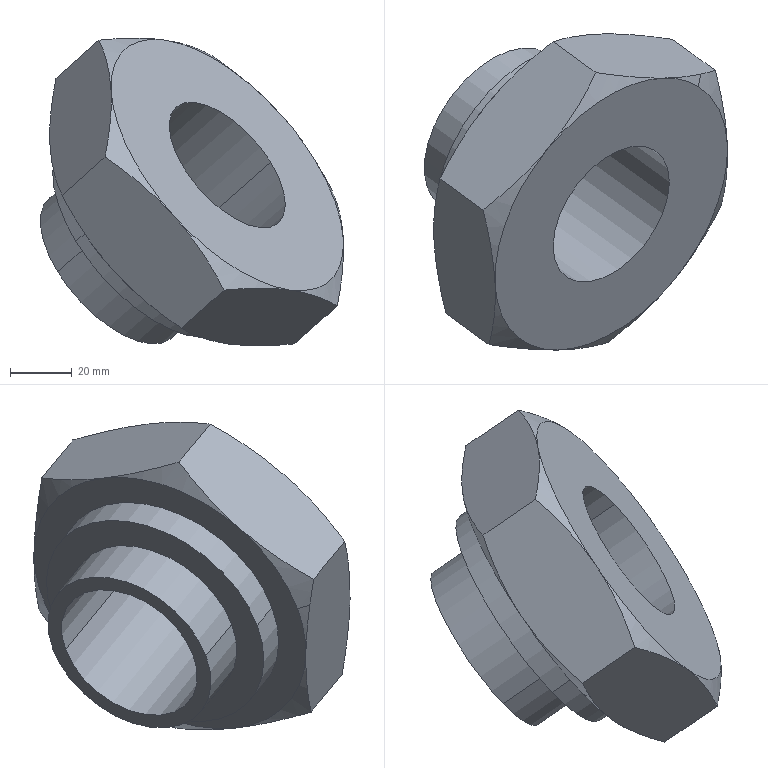Component | SolidWorks | Gasket2-1 | 1 solid | 30 faces | box 98.1 x 102.24 x 99.49 mm | volume 244481 mm3 | cone 14 | plane 10 | cylinder 6 | commonest cylinder face diameters 60 x2 50 x2 80 x2 | material Copper
STEP:
#1=COLOUR_RGB('',0.7922,0.8196,0.9333);
#2=FILL_AREA_STYLE_COLOUR('',#1);
#3=FILL_AREA_STYLE('',(#2));
#4=SURFACE_STYLE_FILL_AREA(#3);
#5=SURFACE_SIDE_STYLE('',(#4));
#6=SURFACE_STYLE_USAGE(.BOTH.,#5);
#7=PRESENTATION_STYLE_ASSIGNMENT((#6));
#8=CARTESIAN_POINT('',(6.93,-76.852,19.128));
#9=VERTEX_POINT('',#8);
#10=CARTESIAN_POINT('',(7.298,-77.585,18.111));
#11=VERTEX_POINT('',#10);
#12=CARTESIAN_POINT('',(8.409,-75.962,18.181));
#13=DIRECTION('',(0.6592,-0.4763,0.5818));
#14=DIRECTION('',(0.5643,0.8248,0.03594));
#15=AXIS2_PLACEMENT_3D('',#12,#13,#14);
#16=CIRCLE('',#15,1.969);
#17=EDGE_CURVE('',#9,#11,#16,.T.);
#18=ORIENTED_EDGE('',*,*,#17,.T.);
#19=CARTESIAN_POINT('',(7.272,-77.743,18.154));
#20=VERTEX_POINT('',#19);
#21=CARTESIAN_POINT('',(7.298,-77.585,18.111));
#22=DIRECTION('',(-0.1591,-0.9525,0.2598));
#23=VECTOR('',#22,39.37);
#24=LINE('',#21,#23);
#25=EDGE_CURVE('',#11,#20,#24,.T.);
#26=ORIENTED_EDGE('',*,*,#25,.T.);
#27=CARTESIAN_POINT('',(7.085,-77.793,18.485));
#28=VERTEX_POINT('',#27);
#29=CARTESIAN_POINT('',(7.272,-77.743,18.154));
#30=CARTESIAN_POINT('',(7.206,-77.757,18.262));
#31=CARTESIAN_POINT('',(7.144,-77.774,18.373));
#32=CARTESIAN_POINT('',(7.085,-77.793,18.485));
#33=B_SPLINE_CURVE_WITH_KNOTS('',3,(#29,#30,#31,#32),.UNSPECIFIED.,.F.,.F.,(4,4),(0.04863,0.05831),.UNSPECIFIED.);
#34=EDGE_CURVE('',#20,#28,#33,.T.);
#35=ORIENTED_EDGE('',*,*,#34,.T.);
#36=CARTESIAN_POINT('',(7.085,-77.793,18.485));
#37=CARTESIAN_POINT('',(7.043,-77.627,18.576));
#38=CARTESIAN_POINT('',(7.008,-77.464,18.673));
#39=CARTESIAN_POINT('',(6.968,-77.229,18.832));
#40=CARTESIAN_POINT('',(6.957,-77.151,18.888));
#41=CARTESIAN_POINT('',(6.94,-76.999,19.004));
#42=CARTESIAN_POINT('',(6.934,-76.925,19.065));
#43=CARTESIAN_POINT('',(6.93,-76.852,19.128));
#44=B_SPLINE_CURVE_WITH_KNOTS('',3,(#36,#37,#38,#39,#40,#41,#42,#43),.UNSPECIFIED.,.F.,.F.,(4,2,2,4),(0.00000026,0.0146,0.02191,0.02921),.UNSPECIFIED.);
#45=EDGE_CURVE('',#28,#9,#44,.T.);
#46=ORIENTED_EDGE('',*,*,#45,.T.);
#47=EDGE_LOOP('',(#18,#26,#35,#46));
#48=FACE_OUTER_BOUND('',#47,.T.);
#49=CARTESIAN_POINT('',(8.409,-75.962,18.181));
#50=DIRECTION('',(0.6592,-0.4763,0.5818));
#51=DIRECTION('',(-0.5643,-0.8248,-0.03594));
#52=AXIS2_PLACEMENT_3D('',#49,#50,#51);
#53=CONICAL_SURFACE('',#52,1.969,1.047);
#54=ADVANCED_FACE('',(#48),#53,.T.);
#55=CARTESIAN_POINT('',(10.298,-74.901,18.939));
#56=VERTEX_POINT('',#55);
#57=CARTESIAN_POINT('',(9.869,-74.794,19.513));
#58=VERTEX_POINT('',#57);
#59=CARTESIAN_POINT('',(9.188,-76.524,18.869));
#60=DIRECTION('',(0.6592,-0.4763,0.5818));
#61=DIRECTION('',(0.5643,0.8248,0.03594));
#62=AXIS2_PLACEMENT_3D('',#59,#60,#61);
#63=CIRCLE('',#62,1.969);
#64=EDGE_CURVE('',#56,#58,#63,.T.);
#65=ORIENTED_EDGE('',*,*,#64,.F.);
#66=CARTESIAN_POINT('',(10.325,-74.743,18.896));
#67=VERTEX_POINT('',#66);
#68=CARTESIAN_POINT('',(10.298,-74.901,18.939));
#69=DIRECTION('',(0.1591,0.9525,-0.2598));
#70=VECTOR('',#69,39.37);
#71=LINE('',#68,#70);
#72=EDGE_CURVE('',#56,#67,#71,.T.);
#73=ORIENTED_EDGE('',*,*,#72,.T.);
#74=CARTESIAN_POINT('',(10.325,-74.743,18.896));
#75=CARTESIAN_POINT('',(10.258,-74.758,19.005));
#76=CARTESIAN_POINT('',(10.187,-74.769,19.111));
#77=CARTESIAN_POINT('',(10.036,-74.786,19.317));
#78=CARTESIAN_POINT('',(9.955,-74.792,19.417));
#79=CARTESIAN_POINT('',(9.869,-74.794,19.513));
#80=B_SPLINE_CURVE_WITH_KNOTS('',3,(#74,#75,#76,#77,#78,#79),.UNSPECIFIED.,.F.,.F.,(4,2,4),(0.0097,0.01945,0.02921),.UNSPECIFIED.);
#81=EDGE_CURVE('',#67,#58,#80,.T.);
#82=ORIENTED_EDGE('',*,*,#81,.T.);
#83=EDGE_LOOP('',(#65,#73,#82));
#84=FACE_OUTER_BOUND('',#83,.T.);
#85=CARTESIAN_POINT('',(9.188,-76.524,18.869));
#86=DIRECTION('',(-0.6592,0.4763,-0.5818));
#87=DIRECTION('',(0.5643,0.8248,0.03594));
#88=AXIS2_PLACEMENT_3D('',#85,#86,#87);
#89=CONICAL_SURFACE('',#88,1.969,1.047);
#90=ADVANCED_FACE('',(#84),#89,.T.);
#91=CARTESIAN_POINT('',(7.029,-76.42,17.509));
#92=VERTEX_POINT('',#91);
#93=CARTESIAN_POINT('',(8.362,-74.472,17.594));
#94=VERTEX_POINT('',#93);
#95=CARTESIAN_POINT('',(7.695,-75.446,17.551));
#96=DIRECTION('',(-0.6592,0.4763,-0.5818));
#97=DIRECTION('',(-0.5643,-0.8248,-0.03594));
#98=AXIS2_PLACEMENT_3D('',#95,#96,#97);
#99=CIRCLE('',#98,1.181);
#100=EDGE_CURVE('',#92,#94,#99,.T.);
#101=ORIENTED_EDGE('',*,*,#100,.F.);
#102=CARTESIAN_POINT('',(7.483,-76.748,17.91));
#103=VERTEX_POINT('',#102);
#104=CARTESIAN_POINT('',(7.029,-76.42,17.509));
#105=DIRECTION('',(0.6592,-0.4763,0.5818));
#106=VECTOR('',#105,39.37);
#107=LINE('',#104,#106);
#108=EDGE_CURVE('',#92,#103,#107,.T.);
#109=ORIENTED_EDGE('',*,*,#108,.T.);
#110=CARTESIAN_POINT('',(8.816,-74.8,17.995));
#111=VERTEX_POINT('',#110);
#112=CARTESIAN_POINT('',(8.149,-75.774,17.952));
#113=DIRECTION('',(-0.6592,0.4763,-0.5818));
#114=DIRECTION('',(-0.5643,-0.8248,-0.03594));
#115=AXIS2_PLACEMENT_3D('',#112,#113,#114);
#116=CIRCLE('',#115,1.181);
#117=EDGE_CURVE('',#103,#111,#116,.T.);
#118=ORIENTED_EDGE('',*,*,#117,.T.);
#119=CARTESIAN_POINT('',(8.362,-74.472,17.594));
#120=DIRECTION('',(0.6592,-0.4763,0.5818));
#121=VECTOR('',#120,39.37);
#122=LINE('',#119,#121);
#123=EDGE_CURVE('',#94,#111,#122,.T.);
#124=ORIENTED_EDGE('',*,*,#123,.F.);
#125=EDGE_LOOP('',(#101,#109,#118,#124));
#126=FACE_OUTER_BOUND('',#125,.T.);
#127=CARTESIAN_POINT('',(7.695,-75.446,17.551));
#128=DIRECTION('',(0.6592,-0.4763,0.5818));
#129=DIRECTION('',(0.5643,0.8248,0.03594));
#130=AXIS2_PLACEMENT_3D('',#127,#128,#129);
#131=CYLINDRICAL_SURFACE('',#130,1.181);
#132=ADVANCED_FACE('',(#126),#131,.T.);
#133=CARTESIAN_POINT('',(8.251,-74.634,17.587));
#134=VERTEX_POINT('',#133);
#135=CARTESIAN_POINT('',(7.14,-76.258,17.516));
#136=VERTEX_POINT('',#135);
#137=CARTESIAN_POINT('',(7.695,-75.446,17.551));
#138=DIRECTION('',(-0.6592,0.4763,-0.5818));
#139=DIRECTION('',(-0.5643,-0.8248,-0.03594));
#140=AXIS2_PLACEMENT_3D('',#137,#138,#139);
#141=CIRCLE('',#140,0.9843);
#142=EDGE_CURVE('',#134,#136,#141,.T.);
#143=ORIENTED_EDGE('',*,*,#142,.T.);
#144=CARTESIAN_POINT('',(8.632,-77.336,18.833));
#145=VERTEX_POINT('',#144);
#146=CARTESIAN_POINT('',(7.14,-76.258,17.516));
#147=DIRECTION('',(0.6592,-0.4763,0.5818));
#148=VECTOR('',#147,39.37);
#149=LINE('',#146,#148);
#150=EDGE_CURVE('',#136,#145,#149,.T.);
#151=ORIENTED_EDGE('',*,*,#150,.T.);
#152=CARTESIAN_POINT('',(9.743,-75.712,18.904));
#153=VERTEX_POINT('',#152);
#154=CARTESIAN_POINT('',(9.188,-76.524,18.869));
#155=DIRECTION('',(-0.6592,0.4763,-0.5818));
#156=DIRECTION('',(-0.5643,-0.8248,-0.03594));
#157=AXIS2_PLACEMENT_3D('',#154,#155,#156);
#158=CIRCLE('',#157,0.9843);
#159=EDGE_CURVE('',#153,#145,#158,.T.);
#160=ORIENTED_EDGE('',*,*,#159,.F.);
#161=CARTESIAN_POINT('',(8.251,-74.634,17.587));
#162=DIRECTION('',(0.6592,-0.4763,0.5818));
#163=VECTOR('',#162,39.37);
#164=LINE('',#161,#163);
#165=EDGE_CURVE('',#134,#153,#164,.T.);
#166=ORIENTED_EDGE('',*,*,#165,.F.);
#167=EDGE_LOOP('',(#143,#151,#160,#166));
#168=FACE_OUTER_BOUND('',#167,.T.);
#169=CARTESIAN_POINT('',(7.695,-75.446,17.551));
#170=DIRECTION('',(0.6592,-0.4763,0.5818));
#171=DIRECTION('',(0.5643,0.8248,0.03594));
#172=AXIS2_PLACEMENT_3D('',#169,#170,#171);
#173=CYLINDRICAL_SURFACE('',#172,0.9843);
#174=ADVANCED_FACE('',(#168),#173,.F.);
#175=CARTESIAN_POINT('',(7.261,-77.073,17.896));
#176=VERTEX_POINT('',#175);
#177=CARTESIAN_POINT('',(9.038,-74.475,18.009));
#178=VERTEX_POINT('',#177);
#179=CARTESIAN_POINT('',(8.149,-75.774,17.952));
#180=DIRECTION('',(-0.6592,0.4763,-0.5818));
#181=DIRECTION('',(-0.5643,-0.8248,-0.03594));
#182=AXIS2_PLACEMENT_3D('',#179,#180,#181);
#183=CIRCLE('',#182,1.575);
#184=EDGE_CURVE('',#176,#178,#183,.T.);
#185=ORIENTED_EDGE('',*,*,#184,.F.);
#186=CARTESIAN_POINT('',(7.52,-77.261,18.125));
#187=VERTEX_POINT('',#186);
#188=CARTESIAN_POINT('',(7.261,-77.073,17.896));
#189=DIRECTION('',(0.6592,-0.4763,0.5818));
#190=VECTOR('',#189,39.37);
#191=LINE('',#188,#190);
#192=EDGE_CURVE('',#176,#187,#191,.T.);
#193=ORIENTED_EDGE('',*,*,#192,.T.);
#194=CARTESIAN_POINT('',(9.298,-74.663,18.238));
#195=VERTEX_POINT('',#194);
#196=CARTESIAN_POINT('',(8.409,-75.962,18.181));
#197=DIRECTION('',(0.6592,-0.4763,0.5818));
#198=DIRECTION('',(0.5643,0.8248,0.03594));
#199=AXIS2_PLACEMENT_3D('',#196,#197,#198);
#200=CIRCLE('',#199,1.575);
#201=EDGE_CURVE('',#195,#187,#200,.T.);
#202=ORIENTED_EDGE('',*,*,#201,.F.);
#203=CARTESIAN_POINT('',(9.038,-74.475,18.009));
#204=DIRECTION('',(0.6592,-0.4763,0.5818));
#205=VECTOR('',#204,39.37);
#206=LINE('',#203,#205);
#207=EDGE_CURVE('',#178,#195,#206,.T.);
#208=ORIENTED_EDGE('',*,*,#207,.F.);
#209=EDGE_LOOP('',(#185,#193,#202,#208));
#210=FACE_OUTER_BOUND('',#209,.T.);
#211=CARTESIAN_POINT('',(8.149,-75.774,17.952));
#212=DIRECTION('',(0.6592,-0.4763,0.5818));
#213=DIRECTION('',(0.5643,0.8248,0.03594));
#214=AXIS2_PLACEMENT_3D('',#211,#212,#213);
#215=CYLINDRICAL_SURFACE('',#214,1.575);
#216=ADVANCED_FACE('',(#210),#215,.T.);
#217=CARTESIAN_POINT('',(9.965,-74.298,18.082));
#218=VERTEX_POINT('',#217);
#219=CARTESIAN_POINT('',(9.888,-75.072,17.235));
#220=VERTEX_POINT('',#219);
#221=CARTESIAN_POINT('',(9.965,-74.298,18.082));
#222=CARTESIAN_POINT('',(9.936,-74.413,17.929));
#223=CARTESIAN_POINT('',(9.913,-74.533,17.781));
#224=CARTESIAN_POINT('',(9.892,-74.725,17.568));
#225=CARTESIAN_POINT('',(9.888,-74.791,17.499));
#226=CARTESIAN_POINT('',(9.884,-74.928,17.364));
#227=CARTESIAN_POINT('',(9.884,-74.999,17.298));
#228=CARTESIAN_POINT('',(9.888,-75.072,17.235));
#229=B_SPLINE_CURVE_WITH_KNOTS('',3,(#221,#222,#223,#224,#225,#226,#227,#228),.UNSPECIFIED.,.F.,.F.,(4,2,2,4),(0.00000026,0.0146,0.02191,0.02921),.UNSPECIFIED.);
#230=EDGE_CURVE('',#218,#220,#229,.T.);
#231=ORIENTED_EDGE('',*,*,#230,.F.);
#232=CARTESIAN_POINT('',(10.512,-74.693,18.565));
#233=VERTEX_POINT('',#232);
#234=CARTESIAN_POINT('',(10.628,-74.777,18.667));
#235=DIRECTION('',(-0.6592,0.4763,-0.5818));
#236=VECTOR('',#235,39.37);
#237=LINE('',#234,#236);
#238=EDGE_CURVE('',#233,#218,#237,.T.);
#239=ORIENTED_EDGE('',*,*,#238,.F.);
#240=CARTESIAN_POINT('',(10.666,-75.634,17.922));
#241=VERTEX_POINT('',#240);
#242=CARTESIAN_POINT('',(10.666,-75.634,17.922));
#243=CARTESIAN_POINT('',(10.665,-75.598,17.954));
#244=CARTESIAN_POINT('',(10.662,-75.561,17.985));
#245=CARTESIAN_POINT('',(10.656,-75.486,18.046));
#246=CARTESIAN_POINT('',(10.653,-75.448,18.075));
#247=CARTESIAN_POINT('',(10.64,-75.334,18.163));
#248=CARTESIAN_POINT('',(10.629,-75.257,18.218));
#249=CARTESIAN_POINT('',(10.589,-75.021,18.378));
#250=CARTESIAN_POINT('',(10.553,-74.859,18.475));
#251=CARTESIAN_POINT('',(10.512,-74.693,18.565));
#252=B_SPLINE_CURVE_WITH_KNOTS('',3,(#242,#243,#244,#245,#246,#247,#248,#249,#250,#251),.UNSPECIFIED.,.F.,.F.,(4,2,2,2,4),(0.02921,0.03285,0.03648,0.04376,0.05831),.UNSPECIFIED.);
#253=EDGE_CURVE('',#241,#233,#252,.T.);
#254=ORIENTED_EDGE('',*,*,#253,.F.);
#255=CARTESIAN_POINT('',(10.589,-76.408,17.074));
#256=VERTEX_POINT('',#255);
#257=CARTESIAN_POINT('',(10.589,-76.408,17.074));
#258=CARTESIAN_POINT('',(10.618,-76.293,17.227));
#259=CARTESIAN_POINT('',(10.641,-76.173,17.376));
#260=CARTESIAN_POINT('',(10.661,-75.981,17.589));
#261=CARTESIAN_POINT('',(10.666,-75.915,17.658));
#262=CARTESIAN_POINT('',(10.67,-75.778,17.793));
#263=CARTESIAN_POINT('',(10.67,-75.707,17.858));
#264=CARTESIAN_POINT('',(10.666,-75.634,17.922));
#265=B_SPLINE_CURVE_WITH_KNOTS('',3,(#257,#258,#259,#260,#261,#262,#263,#264),.UNSPECIFIED.,.F.,.F.,(4,2,2,4),(0.00000026,0.0146,0.02191,0.02921),.UNSPECIFIED.);
#266=EDGE_CURVE('',#256,#241,#265,.T.);
#267=ORIENTED_EDGE('',*,*,#266,.F.);
#268=CARTESIAN_POINT('',(10.042,-76.013,16.592));
#269=VERTEX_POINT('',#268);
#270=CARTESIAN_POINT('',(10.705,-76.491,17.176));
#271=DIRECTION('',(-0.6592,0.4763,-0.5818));
#272=VECTOR('',#271,39.37);
#273=LINE('',#270,#272);
#274=EDGE_CURVE('',#256,#269,#273,.T.);
#275=ORIENTED_EDGE('',*,*,#274,.T.);
#276=CARTESIAN_POINT('',(9.888,-75.072,17.235));
#277=CARTESIAN_POINT('',(9.889,-75.108,17.203));
#278=CARTESIAN_POINT('',(9.892,-75.145,17.172));
#279=CARTESIAN_POINT('',(9.898,-75.22,17.111));
#280=CARTESIAN_POINT('',(9.901,-75.258,17.081));
#281=CARTESIAN_POINT('',(9.914,-75.372,16.994));
#282=CARTESIAN_POINT('',(9.925,-75.449,16.938));
#283=CARTESIAN_POINT('',(9.965,-75.685,16.779));
#284=CARTESIAN_POINT('',(10.001,-75.847,16.682));
#285=CARTESIAN_POINT('',(10.042,-76.013,16.592));
#286=B_SPLINE_CURVE_WITH_KNOTS('',3,(#276,#277,#278,#279,#280,#281,#282,#283,#284,#285),.UNSPECIFIED.,.F.,.F.,(4,2,2,2,4),(0.02921,0.03285,0.03648,0.04376,0.05831),.UNSPECIFIED.);
#287=EDGE_CURVE('',#220,#269,#286,.T.);
#288=ORIENTED_EDGE('',*,*,#287,.F.);
#289=EDGE_LOOP('',(#231,#239,#254,#267,#275,#288));
#290=FACE_OUTER_BOUND('',#289,.T.);
#291=CARTESIAN_POINT('',(10.705,-76.491,17.176));
#292=DIRECTION('',(-0.7512,-0.4521,0.481));
#293=DIRECTION('',(-0.03397,0.7541,0.6559));
#294=AXIS2_PLACEMENT_3D('',#291,#292,#293);
#295=PLANE('',#294);
#296=ADVANCED_FACE('',(#290),#295,.F.);
#297=CARTESIAN_POINT('',(8.448,-74.331,19.775));
#298=VERTEX_POINT('',#297);
#299=CARTESIAN_POINT('',(9.09,-74.231,18.826));
#300=VERTEX_POINT('',#299);
#301=CARTESIAN_POINT('',(8.448,-74.331,19.775));
#302=CARTESIAN_POINT('',(8.536,-74.303,19.605));
#303=CARTESIAN_POINT('',(8.632,-74.279,19.44));
#304=CARTESIAN_POINT('',(8.791,-74.253,19.202));
#305=CARTESIAN_POINT('',(8.847,-74.246,19.124));
#306=CARTESIAN_POINT('',(8.964,-74.236,18.972));
#307=CARTESIAN_POINT('',(9.026,-74.232,18.898));
#308=CARTESIAN_POINT('',(9.09,-74.231,18.826));
#309=B_SPLINE_CURVE_WITH_KNOTS('',3,(#301,#302,#303,#304,#305,#306,#307,#308),.UNSPECIFIED.,.F.,.F.,(4,2,2,4),(0.00000022,0.0146,0.02191,0.02921),.UNSPECIFIED.);
#310=EDGE_CURVE('',#298,#300,#309,.T.);
#311=ORIENTED_EDGE('',*,*,#310,.F.);
#312=CARTESIAN_POINT('',(8.994,-74.726,20.257));
#313=VERTEX_POINT('',#312);
#314=CARTESIAN_POINT('',(9.11,-74.81,20.359));
#315=DIRECTION('',(-0.6592,0.4763,-0.5818));
#316=VECTOR('',#315,39.37);
#317=LINE('',#314,#316);
#318=EDGE_CURVE('',#313,#298,#317,.T.);
#319=ORIENTED_EDGE('',*,*,#318,.F.);
#320=CARTESIAN_POINT('',(9.869,-74.794,19.513));
#321=CARTESIAN_POINT('',(9.837,-74.794,19.549));
#322=CARTESIAN_POINT('',(9.804,-74.795,19.585));
#323=CARTESIAN_POINT('',(9.737,-74.794,19.654));
#324=CARTESIAN_POINT('',(9.703,-74.793,19.688));
#325=CARTESIAN_POINT('',(9.599,-74.79,19.788));
#326=CARTESIAN_POINT('',(9.527,-74.785,19.852));
#327=CARTESIAN_POINT('',(9.307,-74.768,20.037));
#328=CARTESIAN_POINT('',(9.154,-74.749,20.15));
#329=CARTESIAN_POINT('',(8.994,-74.726,20.257));
#330=B_SPLINE_CURVE_WITH_KNOTS('',3,(#320,#321,#322,#323,#324,#325,#326,#327,#328,#329),.UNSPECIFIED.,.F.,.F.,(4,2,2,2,4),(0.02921,0.03285,0.03648,0.04376,0.05831),.UNSPECIFIED.);
#331=EDGE_CURVE('',#58,#313,#330,.T.);
#332=ORIENTED_EDGE('',*,*,#331,.F.);
#333=ORIENTED_EDGE('',*,*,#81,.F.);
#334=CARTESIAN_POINT('',(10.512,-74.693,18.565));
#335=CARTESIAN_POINT('',(10.453,-74.712,18.678));
#336=CARTESIAN_POINT('',(10.391,-74.729,18.788));
#337=CARTESIAN_POINT('',(10.325,-74.743,18.896));
#338=B_SPLINE_CURVE_WITH_KNOTS('',3,(#334,#335,#336,#337),.UNSPECIFIED.,.F.,.F.,(4,4),(0.00000022,0.0097),.UNSPECIFIED.);
#339=EDGE_CURVE('',#233,#67,#338,.T.);
#340=ORIENTED_EDGE('',*,*,#339,.F.);
#341=ORIENTED_EDGE('',*,*,#238,.T.);
#342=CARTESIAN_POINT('',(9.09,-74.231,18.826));
#343=CARTESIAN_POINT('',(9.123,-74.23,18.79));
#344=CARTESIAN_POINT('',(9.156,-74.23,18.755));
#345=CARTESIAN_POINT('',(9.223,-74.231,18.685));
#346=CARTESIAN_POINT('',(9.257,-74.231,18.651));
#347=CARTESIAN_POINT('',(9.361,-74.235,18.551));
#348=CARTESIAN_POINT('',(9.432,-74.239,18.487));
#349=CARTESIAN_POINT('',(9.652,-74.257,18.303));
#350=CARTESIAN_POINT('',(9.806,-74.276,18.189));
#351=CARTESIAN_POINT('',(9.965,-74.298,18.082));
#352=B_SPLINE_CURVE_WITH_KNOTS('',3,(#342,#343,#344,#345,#346,#347,#348,#349,#350,#351),.UNSPECIFIED.,.F.,.F.,(4,2,2,2,4),(0.02921,0.03285,0.03648,0.04376,0.05831),.UNSPECIFIED.);
#353=EDGE_CURVE('',#300,#218,#352,.T.);
#354=ORIENTED_EDGE('',*,*,#353,.F.);
#355=EDGE_LOOP('',(#311,#319,#332,#333,#340,#341,#354));
#356=FACE_OUTER_BOUND('',#355,.T.);
#357=CARTESIAN_POINT('',(10.628,-74.777,18.667));
#358=DIRECTION('',(-0.3462,-0.8791,-0.3275));
#359=DIRECTION('',(-0.6675,-0.01449,0.7444));
#360=AXIS2_PLACEMENT_3D('',#357,#358,#359);
#361=PLANE('',#360);
#362=ADVANCED_FACE('',(#356),#361,.F.);
#363=CARTESIAN_POINT('',(7.008,-76.078,19.976));
#364=VERTEX_POINT('',#363);
#365=CARTESIAN_POINT('',(7.612,-75.121,19.773));
#366=VERTEX_POINT('',#365);
#367=CARTESIAN_POINT('',(7.008,-76.078,19.976));
#368=CARTESIAN_POINT('',(7.09,-75.91,19.928));
#369=CARTESIAN_POINT('',(7.179,-75.745,19.886));
#370=CARTESIAN_POINT('',(7.329,-75.505,19.834));
#371=CARTESIAN_POINT('',(7.381,-75.426,19.819));
#372=CARTESIAN_POINT('',(7.492,-75.271,19.792));
#373=CARTESIAN_POINT('',(7.55,-75.196,19.781));
#374=CARTESIAN_POINT('',(7.612,-75.121,19.773));
#375=B_SPLINE_CURVE_WITH_KNOTS('',3,(#367,#368,#369,#370,#371,#372,#373,#374),.UNSPECIFIED.,.F.,.F.,(4,2,2,4),(0.00000021,0.0146,0.02191,0.02921),.UNSPECIFIED.);
#376=EDGE_CURVE('',#364,#366,#375,.T.);
#377=ORIENTED_EDGE('',*,*,#376,.F.);
#378=CARTESIAN_POINT('',(7.554,-76.473,20.458));
#379=VERTEX_POINT('',#378);
#380=CARTESIAN_POINT('',(7.67,-76.557,20.561));
#381=DIRECTION('',(-0.6592,0.4763,-0.5818));
#382=VECTOR('',#381,39.37);
#383=LINE('',#380,#382);
#384=EDGE_CURVE('',#379,#364,#383,.T.);
#385=ORIENTED_EDGE('',*,*,#384,.F.);
#386=CARTESIAN_POINT('',(8.39,-75.684,20.46));
#387=VERTEX_POINT('',#386);
#388=CARTESIAN_POINT('',(8.39,-75.684,20.46));
#389=CARTESIAN_POINT('',(8.36,-75.721,20.464));
#390=CARTESIAN_POINT('',(8.328,-75.758,20.468));
#391=CARTESIAN_POINT('',(8.265,-75.83,20.474));
#392=CARTESIAN_POINT('',(8.232,-75.865,20.477));
#393=CARTESIAN_POINT('',(8.133,-75.97,20.482));
#394=CARTESIAN_POINT('',(8.065,-76.037,20.484));
#395=CARTESIAN_POINT('',(7.855,-76.234,20.482));
#396=CARTESIAN_POINT('',(7.707,-76.356,20.473));
#397=CARTESIAN_POINT('',(7.554,-76.473,20.458));
#398=B_SPLINE_CURVE_WITH_KNOTS('',3,(#388,#389,#390,#391,#392,#393,#394,#395,#396,#397),.UNSPECIFIED.,.F.,.F.,(4,2,2,2,4),(0.02921,0.03285,0.03648,0.04376,0.05831),.UNSPECIFIED.);
#399=EDGE_CURVE('',#387,#379,#398,.T.);
#400=ORIENTED_EDGE('',*,*,#399,.F.);
#401=CARTESIAN_POINT('',(8.994,-74.726,20.257));
#402=CARTESIAN_POINT('',(8.912,-74.895,20.305));
#403=CARTESIAN_POINT('',(8.823,-75.06,20.347));
#404=CARTESIAN_POINT('',(8.673,-75.3,20.399));
#405=CARTESIAN_POINT('',(8.621,-75.379,20.414));
#406=CARTESIAN_POINT('',(8.51,-75.533,20.441));
#407=CARTESIAN_POINT('',(8.452,-75.609,20.452));
#408=CARTESIAN_POINT('',(8.39,-75.684,20.46));
#409=B_SPLINE_CURVE_WITH_KNOTS('',3,(#401,#402,#403,#404,#405,#406,#407,#408),.UNSPECIFIED.,.F.,.F.,(4,2,2,4),(0.00000021,0.0146,0.02191,0.02921),.UNSPECIFIED.);
#410=EDGE_CURVE('',#313,#387,#409,.T.);
#411=ORIENTED_EDGE('',*,*,#410,.F.);
#412=ORIENTED_EDGE('',*,*,#318,.T.);
#413=CARTESIAN_POINT('',(7.612,-75.121,19.773));
#414=CARTESIAN_POINT('',(7.642,-75.084,19.769));
#415=CARTESIAN_POINT('',(7.674,-75.047,19.765));
#416=CARTESIAN_POINT('',(7.737,-74.975,19.759));
#417=CARTESIAN_POINT('',(7.77,-74.94,19.756));
#418=CARTESIAN_POINT('',(7.869,-74.835,19.751));
#419=CARTESIAN_POINT('',(7.937,-74.767,19.749));
#420=CARTESIAN_POINT('',(8.147,-74.571,19.751));
#421=CARTESIAN_POINT('',(8.295,-74.448,19.76));
#422=CARTESIAN_POINT('',(8.448,-74.331,19.775));
#423=B_SPLINE_CURVE_WITH_KNOTS('',3,(#413,#414,#415,#416,#417,#418,#419,#420,#421,#422),.UNSPECIFIED.,.F.,.F.,(4,2,2,2,4),(0.02921,0.03285,0.03648,0.04376,0.05831),.UNSPECIFIED.);
#424=EDGE_CURVE('',#366,#298,#423,.T.);
#425=ORIENTED_EDGE('',*,*,#424,.F.);
#426=EDGE_LOOP('',(#377,#385,#400,#411,#412,#425));
#427=FACE_OUTER_BOUND('',#426,.T.);
#428=CARTESIAN_POINT('',(9.11,-74.81,20.359));
#429=DIRECTION('',(0.405,-0.427,-0.8085));
#430=DIRECTION('',(-0.6336,-0.7686,0.08859));
#431=AXIS2_PLACEMENT_3D('',#428,#429,#430);
#432=PLANE('',#431);
#433=ADVANCED_FACE('',(#427),#432,.F.);
#434=ORIENTED_EDGE('',*,*,#45,.F.);
#435=CARTESIAN_POINT('',(7.632,-78.188,18.968));
#436=VERTEX_POINT('',#435);
#437=CARTESIAN_POINT('',(7.747,-78.271,19.07));
#438=DIRECTION('',(-0.6592,0.4763,-0.5818));
#439=VECTOR('',#438,39.37);
#440=LINE('',#437,#439);
#441=EDGE_CURVE('',#436,#28,#440,.T.);
#442=ORIENTED_EDGE('',*,*,#441,.F.);
#443=CARTESIAN_POINT('',(7.709,-77.414,19.815));
#444=VERTEX_POINT('',#443);
#445=CARTESIAN_POINT('',(7.709,-77.414,19.815));
#446=CARTESIAN_POINT('',(7.71,-77.451,19.784));
#447=CARTESIAN_POINT('',(7.711,-77.487,19.751));
#448=CARTESIAN_POINT('',(7.712,-77.558,19.686));
#449=CARTESIAN_POINT('',(7.712,-77.592,19.652));
#450=CARTESIAN_POINT('',(7.709,-77.695,19.551));
#451=CARTESIAN_POINT('',(7.704,-77.761,19.482));
#452=CARTESIAN_POINT('',(7.683,-77.953,19.269));
#453=CARTESIAN_POINT('',(7.661,-78.073,19.12));
#454=CARTESIAN_POINT('',(7.632,-78.188,18.968));
#455=B_SPLINE_CURVE_WITH_KNOTS('',3,(#445,#446,#447,#448,#449,#450,#451,#452,#453,#454),.UNSPECIFIED.,.F.,.F.,(4,2,2,2,4),(0.02921,0.03285,0.03648,0.04376,0.05831),.UNSPECIFIED.);
#456=EDGE_CURVE('',#444,#436,#455,.T.);
#457=ORIENTED_EDGE('',*,*,#456,.F.);
#458=CARTESIAN_POINT('',(7.554,-76.473,20.458));
#459=CARTESIAN_POINT('',(7.596,-76.639,20.368));
#460=CARTESIAN_POINT('',(7.632,-76.802,20.271));
#461=CARTESIAN_POINT('',(7.671,-77.037,20.111));
#462=CARTESIAN_POINT('',(7.683,-77.115,20.056));
#463=CARTESIAN_POINT('',(7.7,-77.267,19.94));
#464=CARTESIAN_POINT('',(7.706,-77.341,19.879));
#465=CARTESIAN_POINT('',(7.709,-77.414,19.815));
#466=B_SPLINE_CURVE_WITH_KNOTS('',3,(#458,#459,#460,#461,#462,#463,#464,#465),.UNSPECIFIED.,.F.,.F.,(4,2,2,4),(0.00000026,0.0146,0.02191,0.02921),.UNSPECIFIED.);
#467=EDGE_CURVE('',#379,#444,#466,.T.);
#468=ORIENTED_EDGE('',*,*,#467,.F.);
#469=ORIENTED_EDGE('',*,*,#384,.T.);
#470=CARTESIAN_POINT('',(6.93,-76.852,19.128));
#471=CARTESIAN_POINT('',(6.929,-76.815,19.16));
#472=CARTESIAN_POINT('',(6.928,-76.779,19.192));
#473=CARTESIAN_POINT('',(6.927,-76.708,19.258));
#474=CARTESIAN_POINT('',(6.927,-76.674,19.291));
#475=CARTESIAN_POINT('',(6.931,-76.571,19.392));
#476=CARTESIAN_POINT('',(6.935,-76.505,19.462));
#477=CARTESIAN_POINT('',(6.956,-76.313,19.675));
#478=CARTESIAN_POINT('',(6.979,-76.193,19.823));
#479=CARTESIAN_POINT('',(7.008,-76.078,19.976));
#480=B_SPLINE_CURVE_WITH_KNOTS('',3,(#470,#471,#472,#473,#474,#475,#476,#477,#478,#479),.UNSPECIFIED.,.F.,.F.,(4,2,2,2,4),(0.02921,0.03285,0.03648,0.04376,0.05831),.UNSPECIFIED.);
#481=EDGE_CURVE('',#9,#364,#480,.T.);
#482=ORIENTED_EDGE('',*,*,#481,.F.);
#483=EDGE_LOOP('',(#434,#442,#457,#468,#469,#482));
#484=FACE_OUTER_BOUND('',#483,.T.);
#485=CARTESIAN_POINT('',(7.67,-76.557,20.561));
#486=DIRECTION('',(0.7512,0.4521,-0.481));
#487=DIRECTION('',(0.03397,-0.7541,-0.6559));
#488=AXIS2_PLACEMENT_3D('',#485,#486,#487);
#489=PLANE('',#488);
#490=ADVANCED_FACE('',(#484),#489,.F.);
#491=CARTESIAN_POINT('',(8.602,-77.76,16.793));
#492=VERTEX_POINT('',#491);
#493=CARTESIAN_POINT('',(7.728,-77.692,17.537));
#494=VERTEX_POINT('',#493);
#495=CARTESIAN_POINT('',(8.602,-77.76,16.793));
#496=CARTESIAN_POINT('',(8.443,-77.737,16.9));
#497=CARTESIAN_POINT('',(8.288,-77.718,17.014));
#498=CARTESIAN_POINT('',(8.069,-77.701,17.198));
#499=CARTESIAN_POINT('',(7.997,-77.696,17.262));
#500=CARTESIAN_POINT('',(7.859,-77.691,17.395));
#501=CARTESIAN_POINT('',(7.792,-77.691,17.465));
#502=CARTESIAN_POINT('',(7.728,-77.692,17.537));
#503=B_SPLINE_CURVE_WITH_KNOTS('',3,(#495,#496,#497,#498,#499,#500,#501,#502),.UNSPECIFIED.,.F.,.F.,(4,2,2,4),(0.00000022,0.0146,0.02191,0.02921),.UNSPECIFIED.);
#504=EDGE_CURVE('',#492,#494,#503,.T.);
#505=ORIENTED_EDGE('',*,*,#504,.F.);
#506=CARTESIAN_POINT('',(9.149,-78.155,17.276));
#507=VERTEX_POINT('',#506);
#508=CARTESIAN_POINT('',(9.265,-78.238,17.378));
#509=DIRECTION('',(-0.6592,0.4763,-0.5818));
#510=VECTOR('',#509,39.37);
#511=LINE('',#508,#510);
#512=EDGE_CURVE('',#507,#492,#511,.T.);
#513=ORIENTED_EDGE('',*,*,#512,.F.);
#514=CARTESIAN_POINT('',(8.506,-78.255,18.224));
#515=VERTEX_POINT('',#514);
#516=CARTESIAN_POINT('',(8.506,-78.255,18.224));
#517=CARTESIAN_POINT('',(8.538,-78.254,18.188));
#518=CARTESIAN_POINT('',(8.57,-78.253,18.151));
#519=CARTESIAN_POINT('',(8.632,-78.25,18.077));
#520=CARTESIAN_POINT('',(8.662,-78.247,18.04));
#521=CARTESIAN_POINT('',(8.75,-78.24,17.926));
#522=CARTESIAN_POINT('',(8.805,-78.233,17.848));
#523=CARTESIAN_POINT('',(8.965,-78.207,17.61));
#524=CARTESIAN_POINT('',(9.06,-78.183,17.445));
#525=CARTESIAN_POINT('',(9.149,-78.155,17.276));
#526=B_SPLINE_CURVE_WITH_KNOTS('',3,(#516,#517,#518,#519,#520,#521,#522,#523,#524,#525),.UNSPECIFIED.,.F.,.F.,(4,2,2,2,4),(0.02921,0.03285,0.03648,0.04376,0.05831),.UNSPECIFIED.);
#527=EDGE_CURVE('',#515,#507,#526,.T.);
#528=ORIENTED_EDGE('',*,*,#527,.F.);
#529=CARTESIAN_POINT('',(7.632,-78.188,18.968));
#530=CARTESIAN_POINT('',(7.791,-78.21,18.861));
#531=CARTESIAN_POINT('',(7.945,-78.229,18.747));
#532=CARTESIAN_POINT('',(8.165,-78.247,18.562));
#533=CARTESIAN_POINT('',(8.236,-78.251,18.498));
#534=CARTESIAN_POINT('',(8.375,-78.256,18.365));
#535=CARTESIAN_POINT('',(8.441,-78.256,18.296));
#536=CARTESIAN_POINT('',(8.506,-78.255,18.224));
#537=B_SPLINE_CURVE_WITH_KNOTS('',3,(#529,#530,#531,#532,#533,#534,#535,#536),.UNSPECIFIED.,.F.,.F.,(4,2,2,4),(0.00000022,0.0146,0.02191,0.02921),.UNSPECIFIED.);
#538=EDGE_CURVE('',#436,#515,#537,.T.);
#539=ORIENTED_EDGE('',*,*,#538,.F.);
#540=ORIENTED_EDGE('',*,*,#441,.T.);
#541=ORIENTED_EDGE('',*,*,#34,.F.);
#542=CARTESIAN_POINT('',(7.728,-77.692,17.537));
#543=CARTESIAN_POINT('',(7.685,-77.693,17.585));
#544=CARTESIAN_POINT('',(7.643,-77.695,17.634));
#545=CARTESIAN_POINT('',(7.562,-77.7,17.734));
#546=CARTESIAN_POINT('',(7.522,-77.704,17.784));
#547=CARTESIAN_POINT('',(7.409,-77.717,17.939));
#548=CARTESIAN_POINT('',(7.338,-77.728,18.045));
#549=CARTESIAN_POINT('',(7.272,-77.743,18.154));
#550=B_SPLINE_CURVE_WITH_KNOTS('',3,(#542,#543,#544,#545,#546,#547,#548,#549),.UNSPECIFIED.,.F.,.F.,(4,2,2,4),(0.02921,0.03406,0.03892,0.04863),.UNSPECIFIED.);
#551=EDGE_CURVE('',#494,#20,#550,.T.);
#552=ORIENTED_EDGE('',*,*,#551,.F.);
#553=EDGE_LOOP('',(#505,#513,#528,#539,#540,#541,#552));
#554=FACE_OUTER_BOUND('',#553,.T.);
#555=CARTESIAN_POINT('',(7.747,-78.271,19.07));
#556=DIRECTION('',(0.3462,0.8791,0.3275));
#557=DIRECTION('',(0.6675,0.01449,-0.7444));
#558=AXIS2_PLACEMENT_3D('',#555,#556,#557);
#559=PLANE('',#558);
#560=ADVANCED_FACE('',(#554),#559,.F.);
#561=CARTESIAN_POINT('',(9.206,-76.802,16.59));
#562=VERTEX_POINT('',#561);
#563=CARTESIAN_POINT('',(10.042,-76.013,16.592));
#564=CARTESIAN_POINT('',(9.889,-76.13,16.577));
#565=CARTESIAN_POINT('',(9.741,-76.253,16.568));
#566=CARTESIAN_POINT('',(9.531,-76.449,16.566));
#567=CARTESIAN_POINT('',(9.463,-76.516,16.568));
#568=CARTESIAN_POINT('',(9.331,-76.656,16.575));
#569=CARTESIAN_POINT('',(9.268,-76.728,16.581));
#570=CARTESIAN_POINT('',(9.206,-76.802,16.59));
#571=B_SPLINE_CURVE_WITH_KNOTS('',3,(#563,#564,#565,#566,#567,#568,#569,#570),.UNSPECIFIED.,.F.,.F.,(4,2,2,4),(0.00000021,0.0146,0.02191,0.02921),.UNSPECIFIED.);
#572=EDGE_CURVE('',#269,#562,#571,.T.);
#573=ORIENTED_EDGE('',*,*,#572,.F.);
#574=ORIENTED_EDGE('',*,*,#274,.F.);
#575=CARTESIAN_POINT('',(9.985,-77.365,17.277));
#576=VERTEX_POINT('',#575);
#577=CARTESIAN_POINT('',(9.985,-77.365,17.277));
#578=CARTESIAN_POINT('',(10.015,-77.328,17.273));
#579=CARTESIAN_POINT('',(10.045,-77.29,17.268));
#580=CARTESIAN_POINT('',(10.104,-77.214,17.257));
#581=CARTESIAN_POINT('',(10.132,-77.176,17.251));
#582=CARTESIAN_POINT('',(10.215,-77.059,17.231));
#583=CARTESIAN_POINT('',(10.268,-76.98,17.216));
#584=CARTESIAN_POINT('',(10.417,-76.74,17.164));
#585=CARTESIAN_POINT('',(10.507,-76.576,17.122));
#586=CARTESIAN_POINT('',(10.589,-76.408,17.074));
#587=B_SPLINE_CURVE_WITH_KNOTS('',3,(#577,#578,#579,#580,#581,#582,#583,#584,#585,#586),.UNSPECIFIED.,.F.,.F.,(4,2,2,2,4),(0.02921,0.03285,0.03648,0.04376,0.05831),.UNSPECIFIED.);
#588=EDGE_CURVE('',#576,#256,#587,.T.);
#589=ORIENTED_EDGE('',*,*,#588,.F.);
#590=CARTESIAN_POINT('',(9.149,-78.155,17.276));
#591=CARTESIAN_POINT('',(9.302,-78.037,17.29));
#592=CARTESIAN_POINT('',(9.45,-77.914,17.299));
#593=CARTESIAN_POINT('',(9.66,-77.718,17.301));
#594=CARTESIAN_POINT('',(9.728,-77.651,17.299));
#595=CARTESIAN_POINT('',(9.86,-77.511,17.292));
#596=CARTESIAN_POINT('',(9.923,-77.439,17.286));
#597=CARTESIAN_POINT('',(9.985,-77.365,17.277));
#598=B_SPLINE_CURVE_WITH_KNOTS('',3,(#590,#591,#592,#593,#594,#595,#596,#597),.UNSPECIFIED.,.F.,.F.,(4,2,2,4),(0.00000021,0.0146,0.02191,0.02921),.UNSPECIFIED.);
#599=EDGE_CURVE('',#507,#576,#598,.T.);
#600=ORIENTED_EDGE('',*,*,#599,.F.);
#601=ORIENTED_EDGE('',*,*,#512,.T.);
#602=CARTESIAN_POINT('',(9.206,-76.802,16.59));
#603=CARTESIAN_POINT('',(9.176,-76.839,16.594));
#604=CARTESIAN_POINT('',(9.146,-76.877,16.599));
#605=CARTESIAN_POINT('',(9.087,-76.953,16.61));
#606=CARTESIAN_POINT('',(9.059,-76.992,16.616));
#607=CARTESIAN_POINT('',(8.976,-77.108,16.636));
#608=CARTESIAN_POINT('',(8.923,-77.187,16.651));
#609=CARTESIAN_POINT('',(8.774,-77.427,16.703));
#610=CARTESIAN_POINT('',(8.684,-77.592,16.745));
#611=CARTESIAN_POINT('',(8.602,-77.76,16.793));
#612=B_SPLINE_CURVE_WITH_KNOTS('',3,(#602,#603,#604,#605,#606,#607,#608,#609,#610,#611),.UNSPECIFIED.,.F.,.F.,(4,2,2,2,4),(0.02921,0.03285,0.03648,0.04376,0.05831),.UNSPECIFIED.);
#613=EDGE_CURVE('',#562,#492,#612,.T.);
#614=ORIENTED_EDGE('',*,*,#613,.F.);
#615=EDGE_LOOP('',(#573,#574,#589,#600,#601,#614));
#616=FACE_OUTER_BOUND('',#615,.T.);
#617=CARTESIAN_POINT('',(9.265,-78.238,17.378));
#618=DIRECTION('',(-0.405,0.427,0.8085));
#619=DIRECTION('',(0.6336,0.7686,-0.08859));
#620=AXIS2_PLACEMENT_3D('',#617,#618,#619);
#621=PLANE('',#620);
#622=ADVANCED_FACE('',(#616),#621,.F.);
#623=ORIENTED_EDGE('',*,*,#201,.T.);
#624=CARTESIAN_POINT('',(8.409,-75.962,18.181));
#625=DIRECTION('',(0.6592,-0.4763,0.5818));
#626=DIRECTION('',(0.5643,0.8248,0.03594));
#627=AXIS2_PLACEMENT_3D('',#624,#625,#626);
#628=CIRCLE('',#627,1.575);
#629=EDGE_CURVE('',#187,#195,#628,.T.);
#630=ORIENTED_EDGE('',*,*,#629,.T.);
#631=EDGE_LOOP('',(#623,#630));
#632=FACE_BOUND('',#631,.T.);
#633=CARTESIAN_POINT('',(8.409,-75.962,18.181));
#634=DIRECTION('',(0.6592,-0.4763,0.5818));
#635=DIRECTION('',(0.5643,0.8248,0.03594));
#636=AXIS2_PLACEMENT_3D('',#633,#634,#635);
#637=CIRCLE('',#636,1.969);
#638=EDGE_CURVE('',#300,#366,#637,.T.);
#639=ORIENTED_EDGE('',*,*,#638,.F.);
#640=CARTESIAN_POINT('',(8.409,-75.962,18.181));
#641=DIRECTION('',(0.6592,-0.4763,0.5818));
#642=DIRECTION('',(0.5643,0.8248,0.03594));
#643=AXIS2_PLACEMENT_3D('',#640,#641,#642);
#644=CIRCLE('',#643,1.969);
#645=EDGE_CURVE('',#220,#300,#644,.T.);
#646=ORIENTED_EDGE('',*,*,#645,.F.);
#647=CARTESIAN_POINT('',(8.409,-75.962,18.181));
#648=DIRECTION('',(0.6592,-0.4763,0.5818));
#649=DIRECTION('',(0.5643,0.8248,0.03594));
#650=AXIS2_PLACEMENT_3D('',#647,#648,#649);
#651=CIRCLE('',#650,1.969);
#652=EDGE_CURVE('',#562,#220,#651,.T.);
#653=ORIENTED_EDGE('',*,*,#652,.F.);
#654=CARTESIAN_POINT('',(8.409,-75.962,18.181));
#655=DIRECTION('',(0.6592,-0.4763,0.5818));
#656=DIRECTION('',(0.5643,0.8248,0.03594));
#657=AXIS2_PLACEMENT_3D('',#654,#655,#656);
#658=CIRCLE('',#657,1.969);
#659=EDGE_CURVE('',#494,#562,#658,.T.);
#660=ORIENTED_EDGE('',*,*,#659,.F.);
#661=CARTESIAN_POINT('',(8.409,-75.962,18.181));
#662=DIRECTION('',(0.6592,-0.4763,0.5818));
#663=DIRECTION('',(0.5643,0.8248,0.03594));
#664=AXIS2_PLACEMENT_3D('',#661,#662,#663);
#665=CIRCLE('',#664,1.969);
#666=EDGE_CURVE('',#11,#494,#665,.T.);
#667=ORIENTED_EDGE('',*,*,#666,.F.);
#668=ORIENTED_EDGE('',*,*,#17,.F.);
#669=CARTESIAN_POINT('',(8.409,-75.962,18.181));
#670=DIRECTION('',(-0.6592,0.4763,-0.5818));
#671=DIRECTION('',(-0.5643,-0.8248,-0.03594));
#672=AXIS2_PLACEMENT_3D('',#669,#670,#671);
#673=CIRCLE('',#672,1.969);
#674=EDGE_CURVE('',#9,#366,#673,.T.);
#675=ORIENTED_EDGE('',*,*,#674,.T.);
#676=EDGE_LOOP('',(#639,#646,#653,#660,#667,#668,#675));
#677=FACE_OUTER_BOUND('',#676,.T.);
#678=CARTESIAN_POINT('',(8.409,-75.962,18.181));
#679=DIRECTION('',(0.6592,-0.4763,0.5818));
#680=DIRECTION('',(0.5643,0.8248,0.03594));
#681=AXIS2_PLACEMENT_3D('',#678,#679,#680);
#682=PLANE('',#681);
#683=ADVANCED_FACE('',(#632,#677),#682,.F.);
#684=ORIENTED_EDGE('',*,*,#159,.T.);
#685=CARTESIAN_POINT('',(9.188,-76.524,18.869));
#686=DIRECTION('',(-0.6592,0.4763,-0.5818));
#687=DIRECTION('',(-0.5643,-0.8248,-0.03594));
#688=AXIS2_PLACEMENT_3D('',#685,#686,#687);
#689=CIRCLE('',#688,0.9843);
#690=EDGE_CURVE('',#145,#153,#689,.T.);
#691=ORIENTED_EDGE('',*,*,#690,.T.);
#692=EDGE_LOOP('',(#684,#691));
#693=FACE_BOUND('',#692,.T.);
#694=CARTESIAN_POINT('',(9.188,-76.524,18.869));
#695=DIRECTION('',(0.6592,-0.4763,0.5818));
#696=DIRECTION('',(0.5643,0.8248,0.03594));
#697=AXIS2_PLACEMENT_3D('',#694,#695,#696);
#698=CIRCLE('',#697,1.969);
#699=EDGE_CURVE('',#241,#56,#698,.T.);
#700=ORIENTED_EDGE('',*,*,#699,.T.);
#701=ORIENTED_EDGE('',*,*,#64,.T.);
#702=CARTESIAN_POINT('',(9.188,-76.524,18.869));
#703=DIRECTION('',(0.6592,-0.4763,0.5818));
#704=DIRECTION('',(0.5643,0.8248,0.03594));
#705=AXIS2_PLACEMENT_3D('',#702,#703,#704);
#706=CIRCLE('',#705,1.969);
#707=EDGE_CURVE('',#58,#387,#706,.T.);
#708=ORIENTED_EDGE('',*,*,#707,.T.);
#709=CARTESIAN_POINT('',(9.188,-76.524,18.869));
#710=DIRECTION('',(0.6592,-0.4763,0.5818));
#711=DIRECTION('',(0.5643,0.8248,0.03594));
#712=AXIS2_PLACEMENT_3D('',#709,#710,#711);
#713=CIRCLE('',#712,1.969);
#714=EDGE_CURVE('',#387,#444,#713,.T.);
#715=ORIENTED_EDGE('',*,*,#714,.T.);
#716=CARTESIAN_POINT('',(9.188,-76.524,18.869));
#717=DIRECTION('',(0.6592,-0.4763,0.5818));
#718=DIRECTION('',(0.5643,0.8248,0.03594));
#719=AXIS2_PLACEMENT_3D('',#716,#717,#718);
#720=CIRCLE('',#719,1.969);
#721=EDGE_CURVE('',#444,#515,#720,.T.);
#722=ORIENTED_EDGE('',*,*,#721,.T.);
#723=CARTESIAN_POINT('',(9.188,-76.524,18.869));
#724=DIRECTION('',(0.6592,-0.4763,0.5818));
#725=DIRECTION('',(0.5643,0.8248,0.03594));
#726=AXIS2_PLACEMENT_3D('',#723,#724,#725);
#727=CIRCLE('',#726,1.969);
#728=EDGE_CURVE('',#515,#576,#727,.T.);
#729=ORIENTED_EDGE('',*,*,#728,.T.);
#730=CARTESIAN_POINT('',(9.188,-76.524,18.869));
#731=DIRECTION('',(0.6592,-0.4763,0.5818));
#732=DIRECTION('',(0.5643,0.8248,0.03594));
#733=AXIS2_PLACEMENT_3D('',#730,#731,#732);
#734=CIRCLE('',#733,1.969);
#735=EDGE_CURVE('',#576,#241,#734,.T.);
#736=ORIENTED_EDGE('',*,*,#735,.T.);
#737=EDGE_LOOP('',(#700,#701,#708,#715,#722,#729,#736));
#738=FACE_OUTER_BOUND('',#737,.T.);
#739=CARTESIAN_POINT('',(9.188,-76.524,18.869));
#740=DIRECTION('',(0.6592,-0.4763,0.5818));
#741=DIRECTION('',(0.5643,0.8248,0.03594));
#742=AXIS2_PLACEMENT_3D('',#739,#740,#741);
#743=PLANE('',#742);
#744=ADVANCED_FACE('',(#693,#738),#743,.T.);
#745=CARTESIAN_POINT('',(8.149,-75.774,17.952));
#746=DIRECTION('',(-0.6592,0.4763,-0.5818));
#747=DIRECTION('',(-0.5643,-0.8248,-0.03594));
#748=AXIS2_PLACEMENT_3D('',#745,#746,#747);
#749=CIRCLE('',#748,1.575);
#750=EDGE_CURVE('',#178,#176,#749,.T.);
#751=ORIENTED_EDGE('',*,*,#750,.T.);
#752=ORIENTED_EDGE('',*,*,#184,.T.);
#753=EDGE_LOOP('',(#751,#752));
#754=FACE_OUTER_BOUND('',#753,.T.);
#755=CARTESIAN_POINT('',(8.149,-75.774,17.952));
#756=DIRECTION('',(-0.6592,0.4763,-0.5818));
#757=DIRECTION('',(-0.5643,-0.8248,-0.03594));
#758=AXIS2_PLACEMENT_3D('',#755,#756,#757);
#759=CIRCLE('',#758,1.181);
#760=EDGE_CURVE('',#111,#103,#759,.T.);
#761=ORIENTED_EDGE('',*,*,#760,.F.);
#762=ORIENTED_EDGE('',*,*,#117,.F.);
#763=EDGE_LOOP('',(#761,#762));
#764=FACE_BOUND('',#763,.T.);
#765=CARTESIAN_POINT('',(8.149,-75.774,17.952));
#766=DIRECTION('',(-0.6592,0.4763,-0.5818));
#767=DIRECTION('',(-0.5643,-0.8248,-0.03594));
#768=AXIS2_PLACEMENT_3D('',#765,#766,#767);
#769=PLANE('',#768);
#770=ADVANCED_FACE('',(#754,#764),#769,.T.);
#771=ORIENTED_EDGE('',*,*,#192,.F.);
#772=ORIENTED_EDGE('',*,*,#750,.F.);
#773=ORIENTED_EDGE('',*,*,#207,.T.);
#774=ORIENTED_EDGE('',*,*,#629,.F.);
#775=EDGE_LOOP('',(#771,#772,#773,#774));
#776=FACE_OUTER_BOUND('',#775,.T.);
#777=CARTESIAN_POINT('',(8.149,-75.774,17.952));
#778=DIRECTION('',(0.6592,-0.4763,0.5818));
#779=DIRECTION('',(0.5643,0.8248,0.03594));
#780=AXIS2_PLACEMENT_3D('',#777,#778,#779);
#781=CYLINDRICAL_SURFACE('',#780,1.575);
#782=ADVANCED_FACE('',(#776),#781,.T.);
#783=ORIENTED_EDGE('',*,*,#150,.F.);
#784=CARTESIAN_POINT('',(7.695,-75.446,17.551));
#785=DIRECTION('',(-0.6592,0.4763,-0.5818));
#786=DIRECTION('',(-0.5643,-0.8248,-0.03594));
#787=AXIS2_PLACEMENT_3D('',#784,#785,#786);
#788=CIRCLE('',#787,0.9843);
#789=EDGE_CURVE('',#136,#134,#788,.T.);
#790=ORIENTED_EDGE('',*,*,#789,.T.);
#791=ORIENTED_EDGE('',*,*,#165,.T.);
#792=ORIENTED_EDGE('',*,*,#690,.F.);
#793=EDGE_LOOP('',(#783,#790,#791,#792));
#794=FACE_OUTER_BOUND('',#793,.T.);
#795=CARTESIAN_POINT('',(7.695,-75.446,17.551));
#796=DIRECTION('',(0.6592,-0.4763,0.5818));
#797=DIRECTION('',(0.5643,0.8248,0.03594));
#798=AXIS2_PLACEMENT_3D('',#795,#796,#797);
#799=CYLINDRICAL_SURFACE('',#798,0.9843);
#800=ADVANCED_FACE('',(#794),#799,.F.);
#801=ORIENTED_EDGE('',*,*,#108,.F.);
#802=CARTESIAN_POINT('',(7.695,-75.446,17.551));
#803=DIRECTION('',(-0.6592,0.4763,-0.5818));
#804=DIRECTION('',(-0.5643,-0.8248,-0.03594));
#805=AXIS2_PLACEMENT_3D('',#802,#803,#804);
#806=CIRCLE('',#805,1.181);
#807=EDGE_CURVE('',#94,#92,#806,.T.);
#808=ORIENTED_EDGE('',*,*,#807,.F.);
#809=ORIENTED_EDGE('',*,*,#123,.T.);
#810=ORIENTED_EDGE('',*,*,#760,.T.);
#811=EDGE_LOOP('',(#801,#808,#809,#810));
#812=FACE_OUTER_BOUND('',#811,.T.);
#813=CARTESIAN_POINT('',(7.695,-75.446,17.551));
#814=DIRECTION('',(0.6592,-0.4763,0.5818));
#815=DIRECTION('',(0.5643,0.8248,0.03594));
#816=AXIS2_PLACEMENT_3D('',#813,#814,#815);
#817=CYLINDRICAL_SURFACE('',#816,1.181);
#818=ADVANCED_FACE('',(#812),#817,.T.);
#819=ORIENTED_EDGE('',*,*,#142,.F.);
#820=ORIENTED_EDGE('',*,*,#789,.F.);
#821=EDGE_LOOP('',(#819,#820));
#822=FACE_BOUND('',#821,.T.);
#823=ORIENTED_EDGE('',*,*,#807,.T.);
#824=ORIENTED_EDGE('',*,*,#100,.T.);
#825=EDGE_LOOP('',(#823,#824));
#826=FACE_OUTER_BOUND('',#825,.T.);
#827=CARTESIAN_POINT('',(7.695,-75.446,17.551));
#828=DIRECTION('',(-0.6592,0.4763,-0.5818));
#829=DIRECTION('',(-0.5643,-0.8248,-0.03594));
#830=AXIS2_PLACEMENT_3D('',#827,#828,#829);
#831=PLANE('',#830);
#832=ADVANCED_FACE('',(#822,#826),#831,.T.);
#833=ORIENTED_EDGE('',*,*,#72,.F.);
#834=ORIENTED_EDGE('',*,*,#699,.F.);
#835=ORIENTED_EDGE('',*,*,#253,.T.);
#836=ORIENTED_EDGE('',*,*,#339,.T.);
#837=EDGE_LOOP('',(#833,#834,#835,#836));
#838=FACE_OUTER_BOUND('',#837,.T.);
#839=CARTESIAN_POINT('',(9.188,-76.524,18.869));
#840=DIRECTION('',(-0.6592,0.4763,-0.5818));
#841=DIRECTION('',(0.5643,0.8248,0.03594));
#842=AXIS2_PLACEMENT_3D('',#839,#840,#841);
#843=CONICAL_SURFACE('',#842,1.969,1.047);
#844=ADVANCED_FACE('',(#838),#843,.T.);
#845=ORIENTED_EDGE('',*,*,#266,.T.);
#846=ORIENTED_EDGE('',*,*,#735,.F.);
#847=ORIENTED_EDGE('',*,*,#588,.T.);
#848=EDGE_LOOP('',(#845,#846,#847));
#849=FACE_OUTER_BOUND('',#848,.T.);
#850=CARTESIAN_POINT('',(9.188,-76.524,18.869));
#851=DIRECTION('',(-0.6592,0.4763,-0.5818));
#852=DIRECTION('',(0.5643,0.8248,0.03594));
#853=AXIS2_PLACEMENT_3D('',#850,#851,#852);
#854=CONICAL_SURFACE('',#853,1.969,1.047);
#855=ADVANCED_FACE('',(#849),#854,.T.);
#856=ORIENTED_EDGE('',*,*,#527,.T.);
#857=ORIENTED_EDGE('',*,*,#599,.T.);
#858=ORIENTED_EDGE('',*,*,#728,.F.);
#859=EDGE_LOOP('',(#856,#857,#858));
#860=FACE_OUTER_BOUND('',#859,.T.);
#861=CARTESIAN_POINT('',(9.188,-76.524,18.869));
#862=DIRECTION('',(-0.6592,0.4763,-0.5818));
#863=DIRECTION('',(0.5643,0.8248,0.03594));
#864=AXIS2_PLACEMENT_3D('',#861,#862,#863);
#865=CONICAL_SURFACE('',#864,1.969,1.047);
#866=ADVANCED_FACE('',(#860),#865,.T.);
#867=ORIENTED_EDGE('',*,*,#456,.T.);
#868=ORIENTED_EDGE('',*,*,#538,.T.);
#869=ORIENTED_EDGE('',*,*,#721,.F.);
#870=EDGE_LOOP('',(#867,#868,#869));
#871=FACE_OUTER_BOUND('',#870,.T.);
#872=CARTESIAN_POINT('',(9.188,-76.524,18.869));
#873=DIRECTION('',(-0.6592,0.4763,-0.5818));
#874=DIRECTION('',(0.5643,0.8248,0.03594));
#875=AXIS2_PLACEMENT_3D('',#872,#873,#874);
#876=CONICAL_SURFACE('',#875,1.969,1.047);
#877=ADVANCED_FACE('',(#871),#876,.T.);
#878=ORIENTED_EDGE('',*,*,#399,.T.);
#879=ORIENTED_EDGE('',*,*,#467,.T.);
#880=ORIENTED_EDGE('',*,*,#714,.F.);
#881=EDGE_LOOP('',(#878,#879,#880));
#882=FACE_OUTER_BOUND('',#881,.T.);
#883=CARTESIAN_POINT('',(9.188,-76.524,18.869));
#884=DIRECTION('',(-0.6592,0.4763,-0.5818));
#885=DIRECTION('',(0.5643,0.8248,0.03594));
#886=AXIS2_PLACEMENT_3D('',#883,#884,#885);
#887=CONICAL_SURFACE('',#886,1.969,1.047);
#888=ADVANCED_FACE('',(#882),#887,.T.);
#889=ORIENTED_EDGE('',*,*,#331,.T.);
#890=ORIENTED_EDGE('',*,*,#410,.T.);
#891=ORIENTED_EDGE('',*,*,#707,.F.);
#892=EDGE_LOOP('',(#889,#890,#891));
#893=FACE_OUTER_BOUND('',#892,.T.);
#894=CARTESIAN_POINT('',(9.188,-76.524,18.869));
#895=DIRECTION('',(-0.6592,0.4763,-0.5818));
#896=DIRECTION('',(0.5643,0.8248,0.03594));
#897=AXIS2_PLACEMENT_3D('',#894,#895,#896);
#898=CONICAL_SURFACE('',#897,1.969,1.047);
#899=ADVANCED_FACE('',(#893),#898,.T.);
#900=ORIENTED_EDGE('',*,*,#353,.T.);
#901=ORIENTED_EDGE('',*,*,#230,.T.);
#902=ORIENTED_EDGE('',*,*,#645,.T.);
#903=EDGE_LOOP('',(#900,#901,#902));
#904=FACE_OUTER_BOUND('',#903,.T.);
#905=CARTESIAN_POINT('',(8.409,-75.962,18.181));
#906=DIRECTION('',(0.6592,-0.4763,0.5818));
#907=DIRECTION('',(-0.5643,-0.8248,-0.03594));
#908=AXIS2_PLACEMENT_3D('',#905,#906,#907);
#909=CONICAL_SURFACE('',#908,1.969,1.047);
#910=ADVANCED_FACE('',(#904),#909,.T.);
#911=ORIENTED_EDGE('',*,*,#287,.T.);
#912=ORIENTED_EDGE('',*,*,#572,.T.);
#913=ORIENTED_EDGE('',*,*,#652,.T.);
#914=EDGE_LOOP('',(#911,#912,#913));
#915=FACE_OUTER_BOUND('',#914,.T.);
#916=CARTESIAN_POINT('',(8.409,-75.962,18.181));
#917=DIRECTION('',(0.6592,-0.4763,0.5818));
#918=DIRECTION('',(-0.5643,-0.8248,-0.03594));
#919=AXIS2_PLACEMENT_3D('',#916,#917,#918);
#920=CONICAL_SURFACE('',#919,1.969,1.047);
#921=ADVANCED_FACE('',(#915),#920,.T.);
#922=ORIENTED_EDGE('',*,*,#504,.T.);
#923=ORIENTED_EDGE('',*,*,#659,.T.);
#924=ORIENTED_EDGE('',*,*,#613,.T.);
#925=EDGE_LOOP('',(#922,#923,#924));
#926=FACE_OUTER_BOUND('',#925,.T.);
#927=CARTESIAN_POINT('',(8.409,-75.962,18.181));
#928=DIRECTION('',(0.6592,-0.4763,0.5818));
#929=DIRECTION('',(-0.5643,-0.8248,-0.03594));
#930=AXIS2_PLACEMENT_3D('',#927,#928,#929);
#931=CONICAL_SURFACE('',#930,1.969,1.047);
#932=ADVANCED_FACE('',(#926),#931,.T.);
#933=ORIENTED_EDGE('',*,*,#25,.F.);
#934=ORIENTED_EDGE('',*,*,#666,.T.);
#935=ORIENTED_EDGE('',*,*,#551,.T.);
#936=EDGE_LOOP('',(#933,#934,#935));
#937=FACE_OUTER_BOUND('',#936,.T.);
#938=CARTESIAN_POINT('',(8.409,-75.962,18.181));
#939=DIRECTION('',(0.6592,-0.4763,0.5818));
#940=DIRECTION('',(-0.5643,-0.8248,-0.03594));
#941=AXIS2_PLACEMENT_3D('',#938,#939,#940);
#942=CONICAL_SURFACE('',#941,1.969,1.047);
#943=ADVANCED_FACE('',(#937),#942,.T.);
#944=ORIENTED_EDGE('',*,*,#376,.T.);
#945=ORIENTED_EDGE('',*,*,#674,.F.);
#946=ORIENTED_EDGE('',*,*,#481,.T.);
#947=EDGE_LOOP('',(#944,#945,#946));
#948=FACE_OUTER_BOUND('',#947,.T.);
#949=CARTESIAN_POINT('',(8.409,-75.962,18.181));
#950=DIRECTION('',(0.6592,-0.4763,0.5818));
#951=DIRECTION('',(-0.5643,-0.8248,-0.03594));
#952=AXIS2_PLACEMENT_3D('',#949,#950,#951);
#953=CONICAL_SURFACE('',#952,1.969,1.047);
#954=ADVANCED_FACE('',(#948),#953,.T.);
#955=ORIENTED_EDGE('',*,*,#424,.T.);
#956=ORIENTED_EDGE('',*,*,#310,.T.);
#957=ORIENTED_EDGE('',*,*,#638,.T.);
#958=EDGE_LOOP('',(#955,#956,#957));
#959=FACE_OUTER_BOUND('',#958,.T.);
#960=CARTESIAN_POINT('',(8.409,-75.962,18.181));
#961=DIRECTION('',(0.6592,-0.4763,0.5818));
#962=DIRECTION('',(-0.5643,-0.8248,-0.03594));
#963=AXIS2_PLACEMENT_3D('',#960,#961,#962);
#964=CONICAL_SURFACE('',#963,1.969,1.047);
#965=ADVANCED_FACE('',(#959),#964,.T.);
#966=CLOSED_SHELL('',(#54,#90,#132,#174,#216,#296,#362,#433,#490,#560,#622,#683,#744,#770,#782,#800,#818,#832,#844,#855,#866,#877,#888,#899,#910,#921,#932,#943,#954,#965));
#967=MANIFOLD_SOLID_BREP('',#966);
#968=STYLED_ITEM('',(#7),#967);
#969=PRESENTATION_LAYER_ASSIGNMENT('','',(#968));
#970=(LENGTH_UNIT()NAMED_UNIT(*)SI_UNIT($,.METRE.));
#971=LENGTH_MEASURE_WITH_UNIT(LENGTH_MEASURE(0.0254),#970);
#972=DIMENSIONAL_EXPONENTS(1.,0.,0.,0.,0.,0.,0.);
#973=(CONVERSION_BASED_UNIT('',#971)LENGTH_UNIT()NAMED_UNIT(#972));
#974=UNCERTAINTY_MEASURE_WITH_UNIT(LENGTH_MEASURE(0.00001),#973,'','');
#975=(NAMED_UNIT(*)PLANE_ANGLE_UNIT()SI_UNIT($,.RADIAN.));
#976=(NAMED_UNIT(*)SI_UNIT($,.STERADIAN.)SOLID_ANGLE_UNIT());
#977=(GEOMETRIC_REPRESENTATION_CONTEXT(3)GLOBAL_UNCERTAINTY_ASSIGNED_CONTEXT((#974))GLOBAL_UNIT_ASSIGNED_CONTEXT((#973,#975,#976))REPRESENTATION_CONTEXT('',''));
#978=MECHANICAL_DESIGN_GEOMETRIC_PRESENTATION_REPRESENTATION('',(#968),#977);
#979=CARTESIAN_POINT('',(0.,0.,0.));
#980=DIRECTION('',(0.,0.,1.));
#981=DIRECTION('',(1.,0.,0.));
#982=AXIS2_PLACEMENT_3D('',#979,#980,#981);
#983=(LENGTH_UNIT()NAMED_UNIT(*)SI_UNIT($,.METRE.));
#984=LENGTH_MEASURE_WITH_UNIT(LENGTH_MEASURE(0.0254),#983);
#985=DIMENSIONAL_EXPONENTS(1.,0.,0.,0.,0.,0.,0.);
#986=(CONVERSION_BASED_UNIT('',#984)LENGTH_UNIT()NAMED_UNIT(#985));
#987=UNCERTAINTY_MEASURE_WITH_UNIT(LENGTH_MEASURE(0.00001),#986,'','');
#988=(NAMED_UNIT(*)PLANE_ANGLE_UNIT()SI_UNIT($,.RADIAN.));
#989=(NAMED_UNIT(*)SI_UNIT($,.STERADIAN.)SOLID_ANGLE_UNIT());
#990=(GEOMETRIC_REPRESENTATION_CONTEXT(3)GLOBAL_UNCERTAINTY_ASSIGNED_CONTEXT((#987))GLOBAL_UNIT_ASSIGNED_CONTEXT((#986,#988,#989))REPRESENTATION_CONTEXT('',''));
#991=ADVANCED_BREP_SHAPE_REPRESENTATION('',(#967,#982),#990);